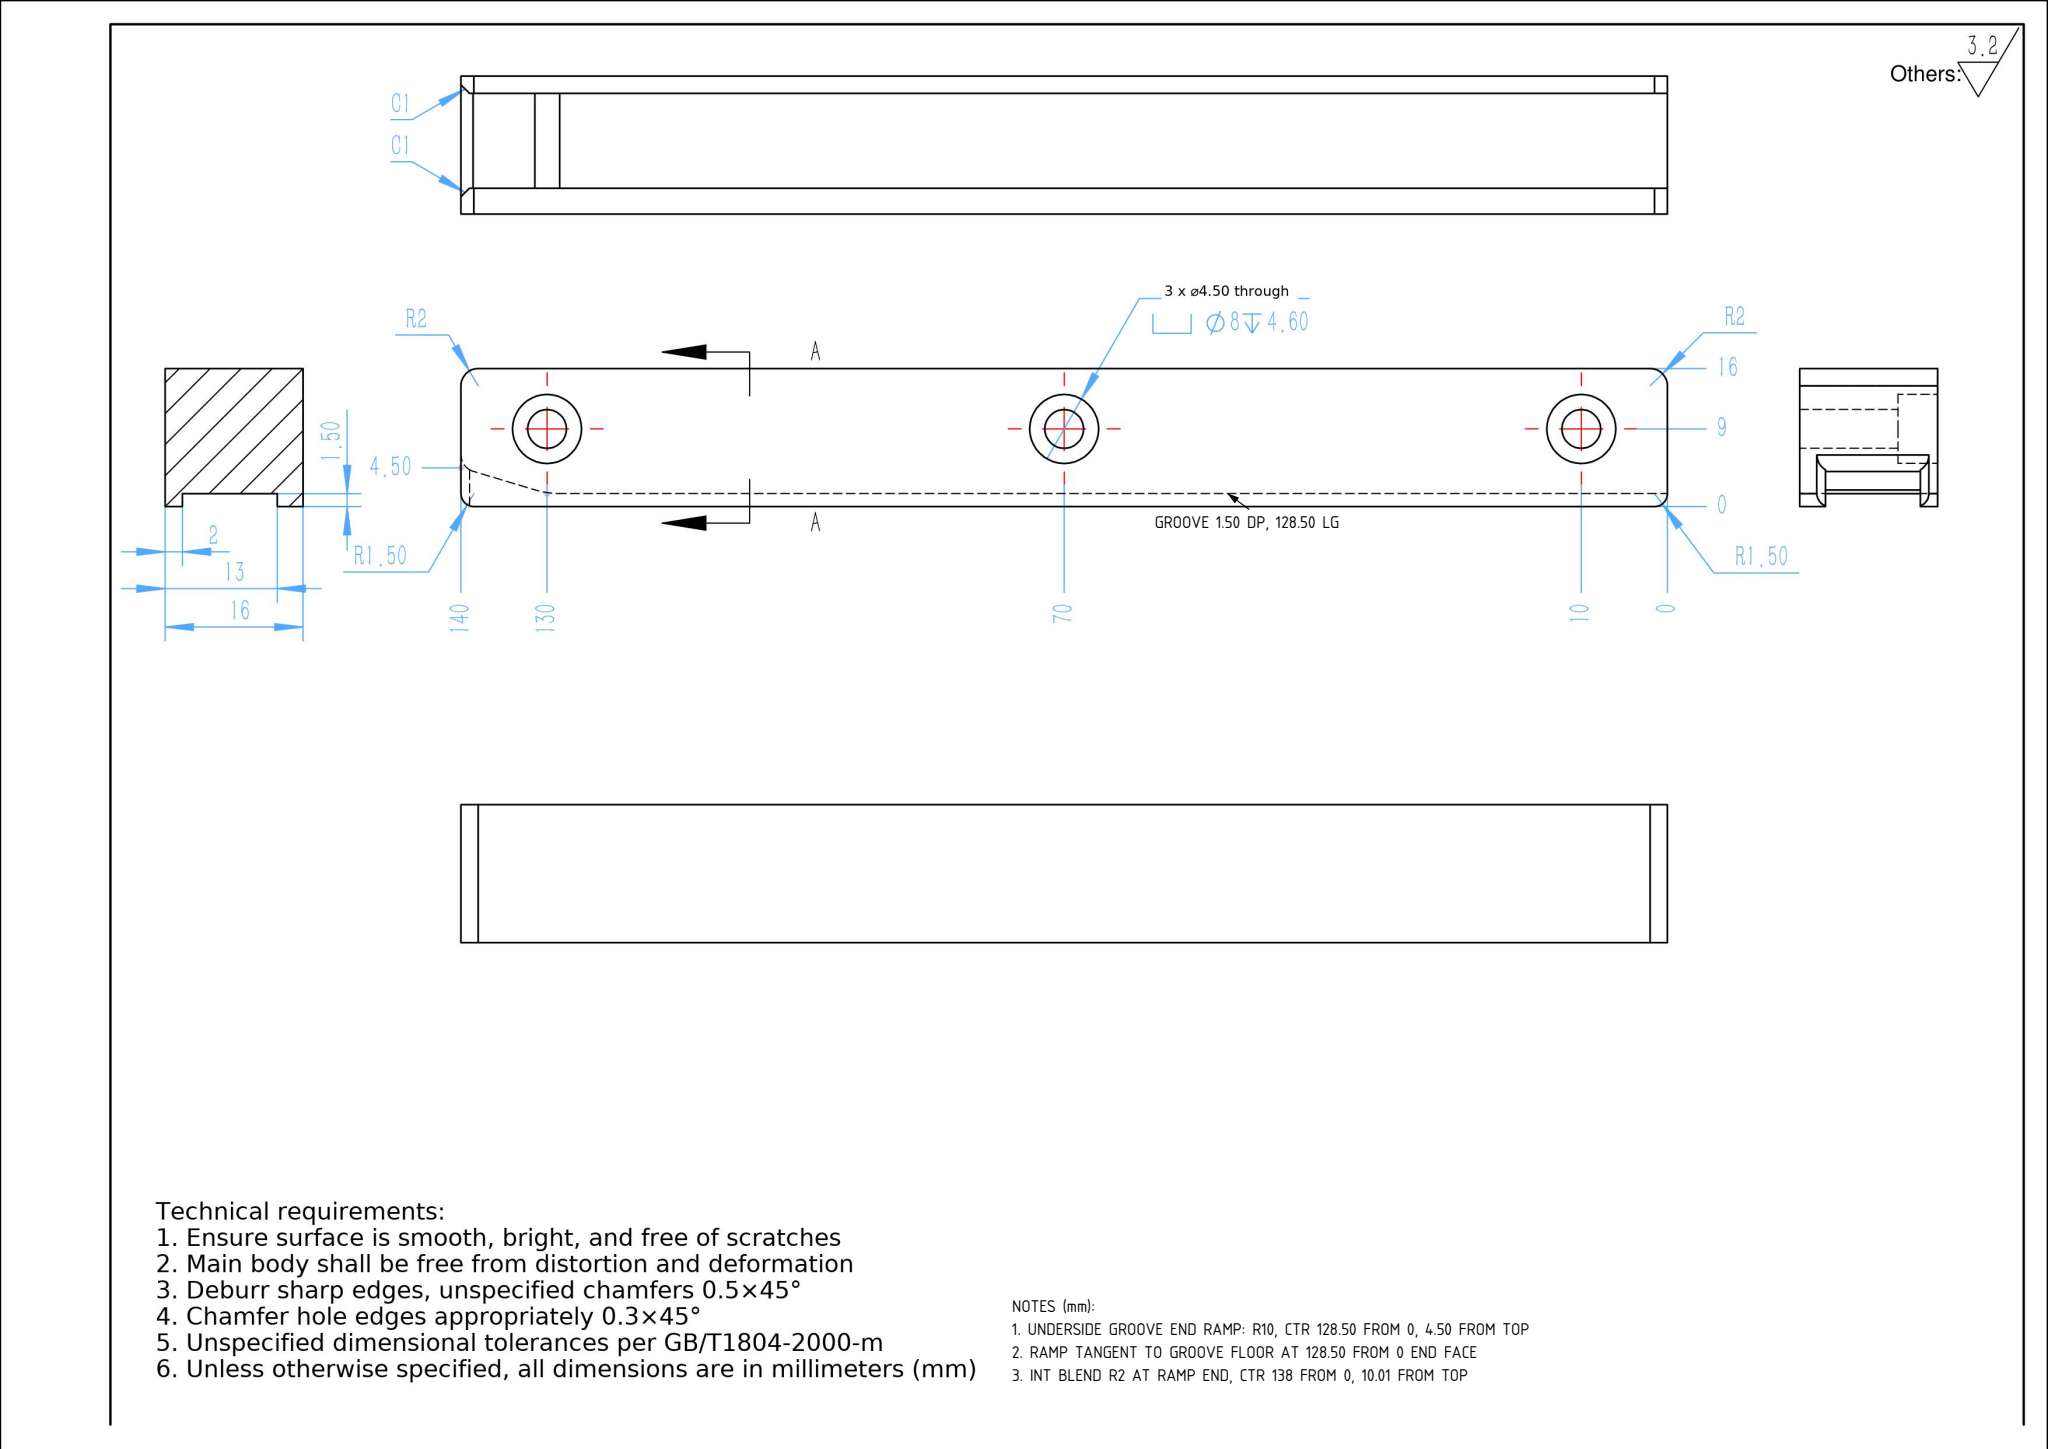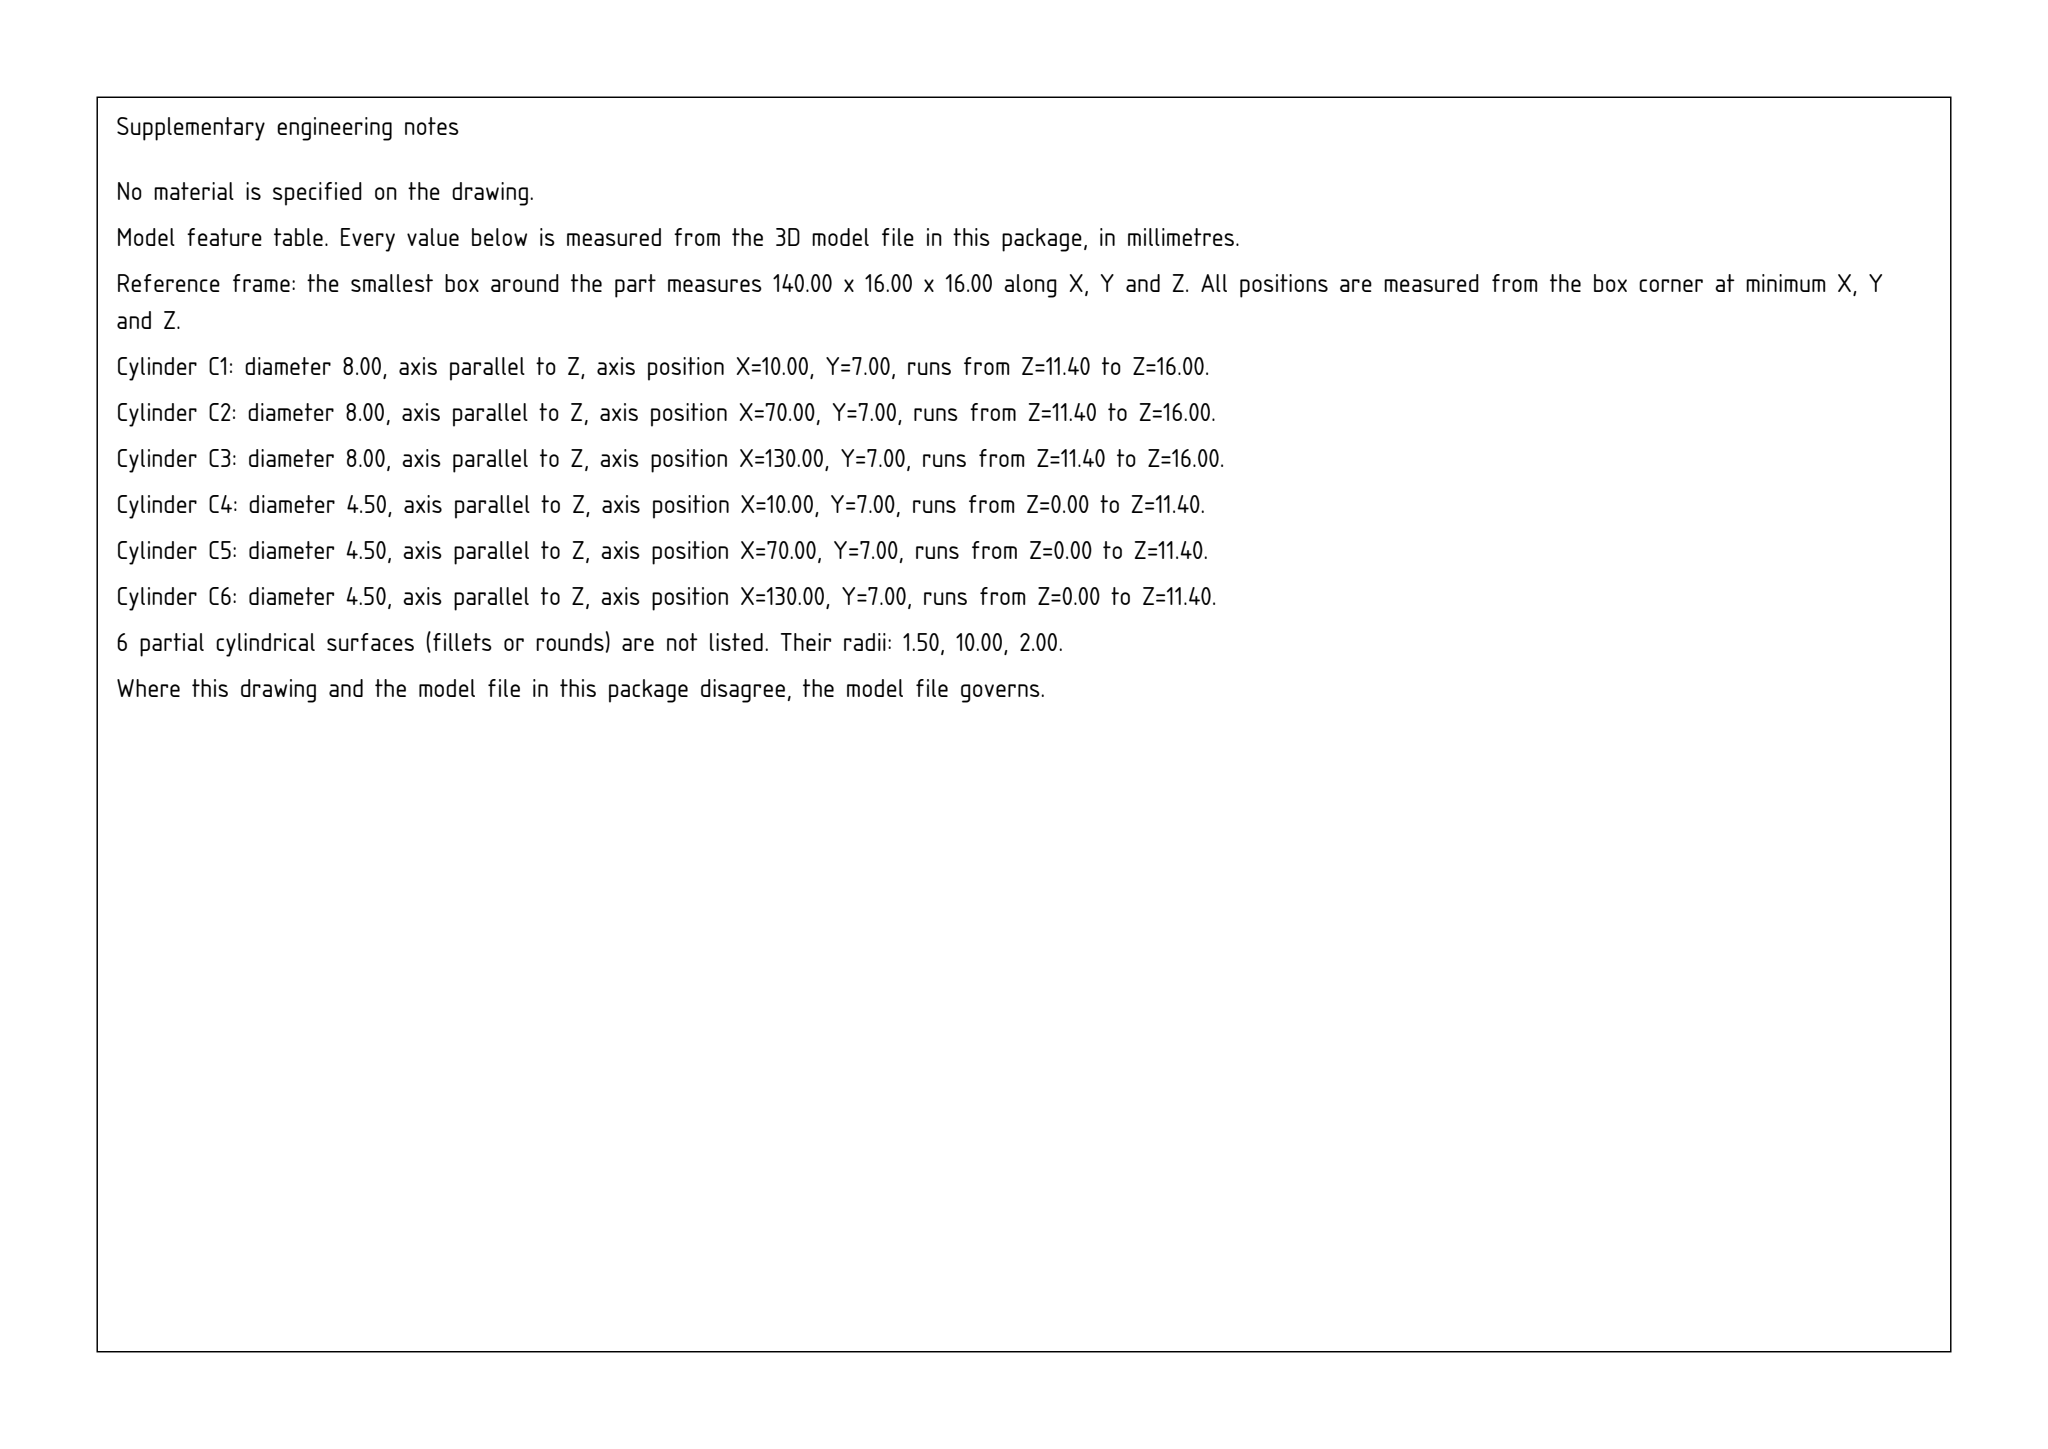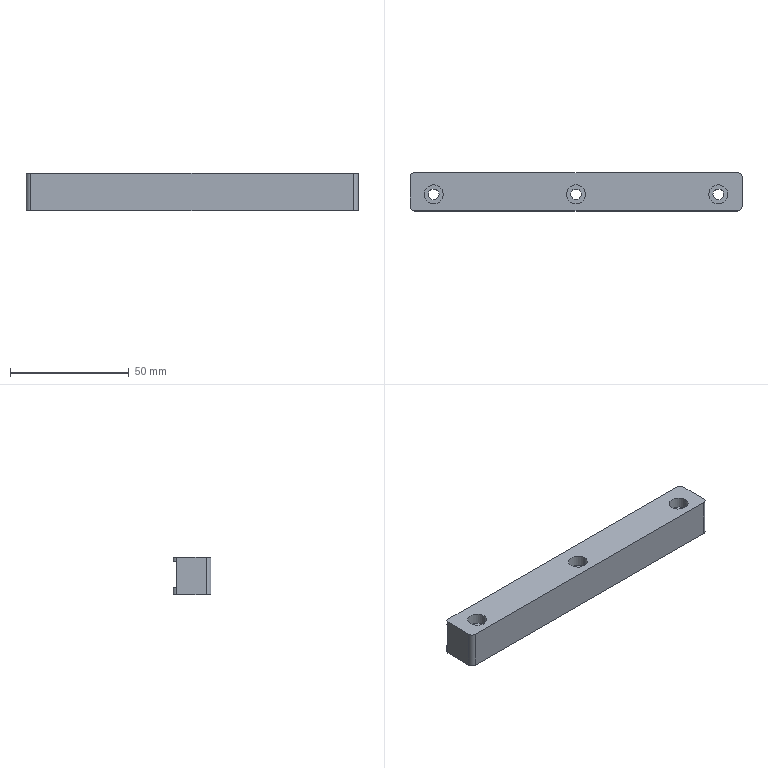Part | SolidWorks | mm | 1 solid | 36 faces | box 140 x 16 x 16 mm | volume 32085 mm3 | cylinder 20 | plane 16 | commonest cylinder face diameters 8 x6 4.5 x6 3 x4 4 x3 20 x1
Drawing notes:
UNDERSIDE GROOVE END RAMP: R10, CTR 128.50 FROM 0, 4.50 FROM TOP | from the solid: cyl dia 20.0 axis z at [x=128.53, y=4.50], len 11.0 (groove width) -> R10 blend arc
RAMP TANGENT TO GROOVE FLOOR AT 128.50 FROM 0 END FACE | from the solid: R10 ctr y=4.50 + R10 = 14.50 = groove floor plane y=14.50; tangent at x=128.53
INT BLEND R2 AT RAMP END, CTR 138 FROM 0, 10.01 FROM TOP | from the solid: cyl dia 4.0 axis z at [x=138.0, y=10.01], len 13.0 -> R2 internal blend, 2 from x=140 face
UNDERSIDE GROOVE 1.50 DP RUNS 0 TO 128.50 FROM 0 END FACE | from the solid: plane y=14.50 (1.50 below y=16 bottom) runs from x=0 end face to R10 tangent x=128.53